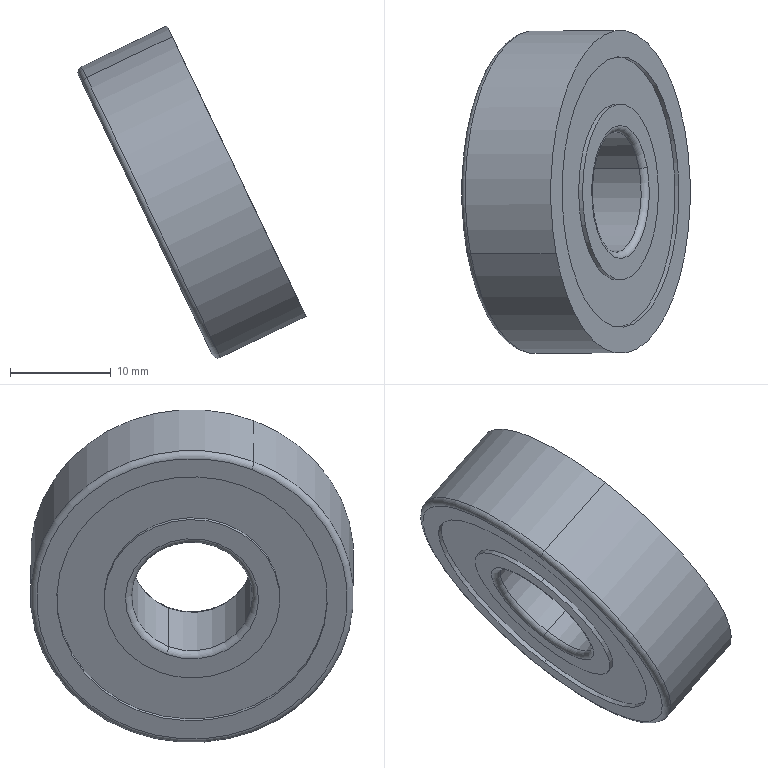Component | SolidWorks | AHTF30S5M100-1_bearingB6201ZZ-1 | 1 solid | 24 faces | volume 6615 mm3 | cylinder 12 | torus 6 | plane 6 | commonest cylinder face diameters 26.8 x4 17.4 x4 12 x2 32 x2
build123d program:
from build123d import *


with BuildPart() as part:
    # Sketch1 → Revolve1 (revolve)
    with BuildSketch(Plane.XY, mode=Mode.PRIVATE) as revolve1_sk:
        with BuildLine():
            Line((0, 16), (0, 13.4))
            Line((0, 13.4), (0.433, 13.4))
            Line((0.433, 13.4), (0.433, 8.7))
            Line((0.433, 8.7), (0, 8.7))
            Line((0, 8.7), (0, 6.6))
            ThreePointArc((0, 6.6), (0.1757, 6.176), (0.6, 6))
            Line((0.6, 6), (9.4, 6))
            ThreePointArc((9.4, 6), (9.824, 6.176), (10, 6.6))
            Line((10, 6.6), (10, 8.7))
            Line((10, 8.7), (9.567, 8.7))
            Line((9.567, 8.7), (9.567, 13.4))
            Line((9.567, 13.4), (10, 13.4))
            Line((10, 13.4), (10, 15.4))
            ThreePointArc((10, 15.4), (9.824, 15.824), (9.4, 16))
            Line((9.4, 16), (0, 16))
        make_face()
    revolve(revolve1_sk.sketch.rotate(Axis((10, 0, 0), (-1, 0, 0)), 270), axis=Axis((10, 0, 0), (-1, 0, 0)))


solid = part.part

# Placed as in the assembly
solid = solid.moved(Location((4.018, 250, 460.302), (47.482, -17.927, -161.443)))
STEP:
#1=COLOUR_RGB('',0.7922,0.8196,0.9333);
#2=FILL_AREA_STYLE_COLOUR('',#1);
#3=FILL_AREA_STYLE('',(#2));
#4=SURFACE_STYLE_FILL_AREA(#3);
#5=SURFACE_SIDE_STYLE('',(#4));
#6=SURFACE_STYLE_USAGE(.BOTH.,#5);
#7=PRESENTATION_STYLE_ASSIGNMENT((#6));
#8=CARTESIAN_POINT('',(0.04487,10.075,17.447));
#9=VERTEX_POINT('',#8);
#10=CARTESIAN_POINT('',(-0.4387,9.61,18.457));
#11=VERTEX_POINT('',#10);
#12=CARTESIAN_POINT('',(-0.1969,9.843,17.952));
#13=DIRECTION('',(0.902,-0.,0.4318));
#14=DIRECTION('',(0.3988,0.3832,-0.8331));
#15=AXIS2_PLACEMENT_3D('',#12,#13,#14);
#16=CIRCLE('',#15,0.6063);
#17=EDGE_CURVE('',#9,#11,#16,.T.);
#18=ORIENTED_EDGE('',*,*,#17,.T.);
#19=CARTESIAN_POINT('',(-0.4269,9.601,18.487));
#20=VERTEX_POINT('',#19);
#21=CARTESIAN_POINT('',(-0.4174,9.61,18.467));
#22=DIRECTION('',(-0.1654,0.9237,0.3456));
#23=DIRECTION('',(0.,-0.3504,0.9366));
#24=AXIS2_PLACEMENT_3D('',#21,#22,#23);
#25=CIRCLE('',#24,0.02362);
#26=EDGE_CURVE('',#11,#20,#25,.T.);
#27=ORIENTED_EDGE('',*,*,#26,.T.);
#28=CARTESIAN_POINT('',(0.0756,10.084,17.438));
#29=VERTEX_POINT('',#28);
#30=CARTESIAN_POINT('',(-0.1756,9.843,17.962));
#31=DIRECTION('',(0.902,-0.,0.4318));
#32=DIRECTION('',(0.3988,0.3832,-0.8331));
#33=AXIS2_PLACEMENT_3D('',#30,#31,#32);
#34=CIRCLE('',#33,0.6299);
#35=EDGE_CURVE('',#29,#20,#34,.T.);
#36=ORIENTED_EDGE('',*,*,#35,.F.);
#37=CARTESIAN_POINT('',(0.06618,10.075,17.457));
#38=DIRECTION('',(0.1654,-0.9237,-0.3456));
#39=DIRECTION('',(0.,0.3504,-0.9366));
#40=AXIS2_PLACEMENT_3D('',#37,#38,#39);
#41=CIRCLE('',#40,0.02362);
#42=EDGE_CURVE('',#9,#29,#41,.T.);
#43=ORIENTED_EDGE('',*,*,#42,.F.);
#44=EDGE_LOOP('',(#18,#27,#36,#43));
#45=FACE_OUTER_BOUND('',#44,.T.);
#46=CARTESIAN_POINT('',(-0.1756,9.843,17.962));
#47=DIRECTION('',(0.902,-0.,0.4318));
#48=DIRECTION('',(0.3988,0.3832,-0.8331));
#49=AXIS2_PLACEMENT_3D('',#46,#47,#48);
#50=TOROIDAL_SURFACE('',#49,0.6063,0.02362);
#51=ADVANCED_FACE('',(#45),#50,.T.);
#52=CARTESIAN_POINT('',(-0.4073,9.64,18.392));
#53=VERTEX_POINT('',#52);
#54=CARTESIAN_POINT('',(0.01347,10.045,17.513));
#55=VERTEX_POINT('',#54);
#56=CARTESIAN_POINT('',(-0.1969,9.843,17.952));
#57=DIRECTION('',(0.902,-0.,0.4318));
#58=DIRECTION('',(0.3988,0.3832,-0.8331));
#59=AXIS2_PLACEMENT_3D('',#56,#57,#58);
#60=CIRCLE('',#59,0.5276);
#61=EDGE_CURVE('',#53,#55,#60,.T.);
#62=ORIENTED_EDGE('',*,*,#61,.F.);
#63=CARTESIAN_POINT('',(-0.392,9.64,18.399));
#64=VERTEX_POINT('',#63);
#65=CARTESIAN_POINT('',(-0.4073,9.64,18.392));
#66=DIRECTION('',(0.902,-0.,0.4318));
#67=VECTOR('',#66,39.37);
#68=LINE('',#65,#67);
#69=EDGE_CURVE('',#53,#64,#68,.T.);
#70=ORIENTED_EDGE('',*,*,#69,.T.);
#71=CARTESIAN_POINT('',(0.02884,10.045,17.52));
#72=VERTEX_POINT('',#71);
#73=CARTESIAN_POINT('',(-0.1816,9.843,17.959));
#74=DIRECTION('',(0.902,-0.,0.4318));
#75=DIRECTION('',(0.3988,0.3832,-0.8331));
#76=AXIS2_PLACEMENT_3D('',#73,#74,#75);
#77=CIRCLE('',#76,0.5276);
#78=EDGE_CURVE('',#64,#72,#77,.T.);
#79=ORIENTED_EDGE('',*,*,#78,.T.);
#80=CARTESIAN_POINT('',(0.01347,10.045,17.513));
#81=DIRECTION('',(0.902,-0.,0.4318));
#82=VECTOR('',#81,39.37);
#83=LINE('',#80,#82);
#84=EDGE_CURVE('',#55,#72,#83,.T.);
#85=ORIENTED_EDGE('',*,*,#84,.F.);
#86=EDGE_LOOP('',(#62,#70,#79,#85));
#87=FACE_OUTER_BOUND('',#86,.T.);
#88=CARTESIAN_POINT('',(-0.1969,9.843,17.952));
#89=DIRECTION('',(0.902,-0.,0.4318));
#90=DIRECTION('',(0.3988,0.3832,-0.8331));
#91=AXIS2_PLACEMENT_3D('',#88,#89,#90);
#92=CYLINDRICAL_SURFACE('',#91,0.5276);
#93=ADVANCED_FACE('',(#87),#92,.F.);
#94=CARTESIAN_POINT('',(-0.06033,9.974,17.667));
#95=VERTEX_POINT('',#94);
#96=CARTESIAN_POINT('',(-0.3335,9.711,18.237));
#97=VERTEX_POINT('',#96);
#98=CARTESIAN_POINT('',(-0.1969,9.843,17.952));
#99=DIRECTION('',(0.902,-0.,0.4318));
#100=DIRECTION('',(0.3988,0.3832,-0.8331));
#101=AXIS2_PLACEMENT_3D('',#98,#99,#100);
#102=CIRCLE('',#101,0.3425);
#103=EDGE_CURVE('',#95,#97,#102,.T.);
#104=ORIENTED_EDGE('',*,*,#103,.T.);
#105=CARTESIAN_POINT('',(-0.3182,9.711,18.245));
#106=VERTEX_POINT('',#105);
#107=CARTESIAN_POINT('',(-0.3335,9.711,18.237));
#108=DIRECTION('',(0.902,-0.,0.4318));
#109=VECTOR('',#108,39.37);
#110=LINE('',#107,#109);
#111=EDGE_CURVE('',#97,#106,#110,.T.);
#112=ORIENTED_EDGE('',*,*,#111,.T.);
#113=CARTESIAN_POINT('',(-0.04496,9.974,17.674));
#114=VERTEX_POINT('',#113);
#115=CARTESIAN_POINT('',(-0.1816,9.843,17.959));
#116=DIRECTION('',(0.902,-0.,0.4318));
#117=DIRECTION('',(0.3988,0.3832,-0.8331));
#118=AXIS2_PLACEMENT_3D('',#115,#116,#117);
#119=CIRCLE('',#118,0.3425);
#120=EDGE_CURVE('',#114,#106,#119,.T.);
#121=ORIENTED_EDGE('',*,*,#120,.F.);
#122=CARTESIAN_POINT('',(-0.06033,9.974,17.667));
#123=DIRECTION('',(0.902,-0.,0.4318));
#124=VECTOR('',#123,39.37);
#125=LINE('',#122,#124);
#126=EDGE_CURVE('',#95,#114,#125,.T.);
#127=ORIENTED_EDGE('',*,*,#126,.F.);
#128=EDGE_LOOP('',(#104,#112,#121,#127));
#129=FACE_OUTER_BOUND('',#128,.T.);
#130=CARTESIAN_POINT('',(-0.1969,9.843,17.952));
#131=DIRECTION('',(0.902,-0.,0.4318));
#132=DIRECTION('',(0.3988,0.3832,-0.8331));
#133=AXIS2_PLACEMENT_3D('',#130,#131,#132);
#134=CYLINDRICAL_SURFACE('',#133,0.3425);
#135=ADVANCED_FACE('',(#129),#134,.T.);
#136=CARTESIAN_POINT('',(-0.08142,9.933,17.766));
#137=VERTEX_POINT('',#136);
#138=CARTESIAN_POINT('',(-0.2698,9.752,18.159));
#139=VERTEX_POINT('',#138);
#140=CARTESIAN_POINT('',(-0.1756,9.843,17.962));
#141=DIRECTION('',(0.902,-0.,0.4318));
#142=DIRECTION('',(0.3988,0.3832,-0.8331));
#143=AXIS2_PLACEMENT_3D('',#140,#141,#142);
#144=CIRCLE('',#143,0.2362);
#145=EDGE_CURVE('',#137,#139,#144,.T.);
#146=ORIENTED_EDGE('',*,*,#145,.T.);
#147=CARTESIAN_POINT('',(-0.3006,9.743,18.169));
#148=VERTEX_POINT('',#147);
#149=CARTESIAN_POINT('',(-0.2793,9.743,18.179));
#150=DIRECTION('',(-0.1654,0.9237,0.3456));
#151=DIRECTION('',(0.,-0.3504,0.9366));
#152=AXIS2_PLACEMENT_3D('',#149,#150,#151);
#153=CIRCLE('',#152,0.02362);
#154=EDGE_CURVE('',#139,#148,#153,.T.);
#155=ORIENTED_EDGE('',*,*,#154,.T.);
#156=CARTESIAN_POINT('',(-0.09331,9.942,17.736));
#157=VERTEX_POINT('',#156);
#158=CARTESIAN_POINT('',(-0.1969,9.843,17.952));
#159=DIRECTION('',(0.902,-0.,0.4318));
#160=DIRECTION('',(0.3988,0.3832,-0.8331));
#161=AXIS2_PLACEMENT_3D('',#158,#159,#160);
#162=CIRCLE('',#161,0.2598);
#163=EDGE_CURVE('',#157,#148,#162,.T.);
#164=ORIENTED_EDGE('',*,*,#163,.F.);
#165=CARTESIAN_POINT('',(-0.072,9.942,17.746));
#166=DIRECTION('',(0.1654,-0.9237,-0.3456));
#167=DIRECTION('',(0.,0.3504,-0.9366));
#168=AXIS2_PLACEMENT_3D('',#165,#166,#167);
#169=CIRCLE('',#168,0.02362);
#170=EDGE_CURVE('',#137,#157,#169,.T.);
#171=ORIENTED_EDGE('',*,*,#170,.F.);
#172=EDGE_LOOP('',(#146,#155,#164,#171));
#173=FACE_OUTER_BOUND('',#172,.T.);
#174=CARTESIAN_POINT('',(-0.1756,9.843,17.962));
#175=DIRECTION('',(0.902,-0.,0.4318));
#176=DIRECTION('',(0.3988,0.3832,-0.8331));
#177=AXIS2_PLACEMENT_3D('',#174,#175,#176);
#178=TOROIDAL_SURFACE('',#177,0.2598,0.02362);
#179=ADVANCED_FACE('',(#173),#178,.T.);
#180=CARTESIAN_POINT('',(-0.1756,9.843,17.962));
#181=DIRECTION('',(0.902,-0.,0.4318));
#182=DIRECTION('',(0.3988,0.3832,-0.8331));
#183=AXIS2_PLACEMENT_3D('',#180,#181,#182);
#184=CIRCLE('',#183,0.2362);
#185=EDGE_CURVE('',#139,#137,#184,.T.);
#186=ORIENTED_EDGE('',*,*,#185,.F.);
#187=CARTESIAN_POINT('',(0.04265,9.752,18.309));
#188=VERTEX_POINT('',#187);
#189=CARTESIAN_POINT('',(-0.2912,9.752,18.149));
#190=DIRECTION('',(0.902,-0.,0.4318));
#191=VECTOR('',#190,39.37);
#192=LINE('',#189,#191);
#193=EDGE_CURVE('',#139,#188,#192,.T.);
#194=ORIENTED_EDGE('',*,*,#193,.T.);
#195=CARTESIAN_POINT('',(0.2311,9.933,17.915));
#196=VERTEX_POINT('',#195);
#197=CARTESIAN_POINT('',(0.1369,9.843,18.112));
#198=DIRECTION('',(0.902,-0.,0.4318));
#199=DIRECTION('',(0.3988,0.3832,-0.8331));
#200=AXIS2_PLACEMENT_3D('',#197,#198,#199);
#201=CIRCLE('',#200,0.2362);
#202=EDGE_CURVE('',#188,#196,#201,.T.);
#203=ORIENTED_EDGE('',*,*,#202,.T.);
#204=CARTESIAN_POINT('',(-0.1027,9.933,17.755));
#205=DIRECTION('',(0.902,-0.,0.4318));
#206=VECTOR('',#205,39.37);
#207=LINE('',#204,#206);
#208=EDGE_CURVE('',#137,#196,#207,.T.);
#209=ORIENTED_EDGE('',*,*,#208,.F.);
#210=EDGE_LOOP('',(#186,#194,#203,#209));
#211=FACE_OUTER_BOUND('',#210,.T.);
#212=CARTESIAN_POINT('',(-0.1969,9.843,17.952));
#213=DIRECTION('',(0.902,-0.,0.4318));
#214=DIRECTION('',(0.3988,0.3832,-0.8331));
#215=AXIS2_PLACEMENT_3D('',#212,#213,#214);
#216=CYLINDRICAL_SURFACE('',#215,0.2362);
#217=ADVANCED_FACE('',(#211),#216,.F.);
#218=CARTESIAN_POINT('',(0.2618,9.942,17.906));
#219=VERTEX_POINT('',#218);
#220=CARTESIAN_POINT('',(0.05454,9.743,18.339));
#221=VERTEX_POINT('',#220);
#222=CARTESIAN_POINT('',(0.1582,9.843,18.122));
#223=DIRECTION('',(0.902,-0.,0.4318));
#224=DIRECTION('',(0.3988,0.3832,-0.8331));
#225=AXIS2_PLACEMENT_3D('',#222,#223,#224);
#226=CIRCLE('',#225,0.2598);
#227=EDGE_CURVE('',#219,#221,#226,.T.);
#228=ORIENTED_EDGE('',*,*,#227,.T.);
#229=CARTESIAN_POINT('',(0.03323,9.743,18.328));
#230=DIRECTION('',(-0.1654,0.9237,0.3456));
#231=DIRECTION('',(0.,-0.3504,0.9366));
#232=AXIS2_PLACEMENT_3D('',#229,#230,#231);
#233=CIRCLE('',#232,0.02362);
#234=EDGE_CURVE('',#221,#188,#233,.T.);
#235=ORIENTED_EDGE('',*,*,#234,.T.);
#236=CARTESIAN_POINT('',(0.1369,9.843,18.112));
#237=DIRECTION('',(0.902,-0.,0.4318));
#238=DIRECTION('',(0.3988,0.3832,-0.8331));
#239=AXIS2_PLACEMENT_3D('',#236,#237,#238);
#240=CIRCLE('',#239,0.2362);
#241=EDGE_CURVE('',#196,#188,#240,.T.);
#242=ORIENTED_EDGE('',*,*,#241,.F.);
#243=CARTESIAN_POINT('',(0.2405,9.942,17.895));
#244=DIRECTION('',(0.1654,-0.9237,-0.3456));
#245=DIRECTION('',(0.,0.3504,-0.9366));
#246=AXIS2_PLACEMENT_3D('',#243,#244,#245);
#247=CIRCLE('',#246,0.02362);
#248=EDGE_CURVE('',#219,#196,#247,.T.);
#249=ORIENTED_EDGE('',*,*,#248,.F.);
#250=EDGE_LOOP('',(#228,#235,#242,#249));
#251=FACE_OUTER_BOUND('',#250,.T.);
#252=CARTESIAN_POINT('',(0.1369,9.843,18.112));
#253=DIRECTION('',(0.902,-0.,0.4318));
#254=DIRECTION('',(0.3988,0.3832,-0.8331));
#255=AXIS2_PLACEMENT_3D('',#252,#253,#254);
#256=TOROIDAL_SURFACE('',#255,0.2598,0.02362);
#257=ADVANCED_FACE('',(#251),#256,.T.);
#258=CARTESIAN_POINT('',(0.2794,9.974,17.829));
#259=VERTEX_POINT('',#258);
#260=CARTESIAN_POINT('',(0.006187,9.711,18.4));
#261=VERTEX_POINT('',#260);
#262=CARTESIAN_POINT('',(0.1428,9.843,18.115));
#263=DIRECTION('',(0.902,-0.,0.4318));
#264=DIRECTION('',(0.3988,0.3832,-0.8331));
#265=AXIS2_PLACEMENT_3D('',#262,#263,#264);
#266=CIRCLE('',#265,0.3425);
#267=EDGE_CURVE('',#259,#261,#266,.T.);
#268=ORIENTED_EDGE('',*,*,#267,.T.);
#269=CARTESIAN_POINT('',(0.02156,9.711,18.407));
#270=VERTEX_POINT('',#269);
#271=CARTESIAN_POINT('',(-0.3335,9.711,18.237));
#272=DIRECTION('',(0.902,-0.,0.4318));
#273=VECTOR('',#272,39.37);
#274=LINE('',#271,#273);
#275=EDGE_CURVE('',#261,#270,#274,.T.);
#276=ORIENTED_EDGE('',*,*,#275,.T.);
#277=CARTESIAN_POINT('',(0.2948,9.974,17.837));
#278=VERTEX_POINT('',#277);
#279=CARTESIAN_POINT('',(0.1582,9.843,18.122));
#280=DIRECTION('',(0.902,-0.,0.4318));
#281=DIRECTION('',(0.3988,0.3832,-0.8331));
#282=AXIS2_PLACEMENT_3D('',#279,#280,#281);
#283=CIRCLE('',#282,0.3425);
#284=EDGE_CURVE('',#278,#270,#283,.T.);
#285=ORIENTED_EDGE('',*,*,#284,.F.);
#286=CARTESIAN_POINT('',(-0.06033,9.974,17.667));
#287=DIRECTION('',(0.902,-0.,0.4318));
#288=VECTOR('',#287,39.37);
#289=LINE('',#286,#288);
#290=EDGE_CURVE('',#259,#278,#289,.T.);
#291=ORIENTED_EDGE('',*,*,#290,.F.);
#292=EDGE_LOOP('',(#268,#276,#285,#291));
#293=FACE_OUTER_BOUND('',#292,.T.);
#294=CARTESIAN_POINT('',(-0.1969,9.843,17.952));
#295=DIRECTION('',(0.902,-0.,0.4318));
#296=DIRECTION('',(0.3988,0.3832,-0.8331));
#297=AXIS2_PLACEMENT_3D('',#294,#295,#296);
#298=CYLINDRICAL_SURFACE('',#297,0.3425);
#299=ADVANCED_FACE('',(#293),#298,.T.);
#300=CARTESIAN_POINT('',(-0.06761,9.64,18.554));
#301=VERTEX_POINT('',#300);
#302=CARTESIAN_POINT('',(0.3532,10.045,17.675));
#303=VERTEX_POINT('',#302);
#304=CARTESIAN_POINT('',(0.1428,9.843,18.115));
#305=DIRECTION('',(0.902,-0.,0.4318));
#306=DIRECTION('',(0.3988,0.3832,-0.8331));
#307=AXIS2_PLACEMENT_3D('',#304,#305,#306);
#308=CIRCLE('',#307,0.5276);
#309=EDGE_CURVE('',#301,#303,#308,.T.);
#310=ORIENTED_EDGE('',*,*,#309,.F.);
#311=CARTESIAN_POINT('',(-0.05224,9.64,18.562));
#312=VERTEX_POINT('',#311);
#313=CARTESIAN_POINT('',(-0.4073,9.64,18.392));
#314=DIRECTION('',(0.902,-0.,0.4318));
#315=VECTOR('',#314,39.37);
#316=LINE('',#313,#315);
#317=EDGE_CURVE('',#301,#312,#316,.T.);
#318=ORIENTED_EDGE('',*,*,#317,.T.);
#319=CARTESIAN_POINT('',(0.3686,10.045,17.683));
#320=VERTEX_POINT('',#319);
#321=CARTESIAN_POINT('',(0.1582,9.843,18.122));
#322=DIRECTION('',(0.902,-0.,0.4318));
#323=DIRECTION('',(0.3988,0.3832,-0.8331));
#324=AXIS2_PLACEMENT_3D('',#321,#322,#323);
#325=CIRCLE('',#324,0.5276);
#326=EDGE_CURVE('',#312,#320,#325,.T.);
#327=ORIENTED_EDGE('',*,*,#326,.T.);
#328=CARTESIAN_POINT('',(0.01347,10.045,17.513));
#329=DIRECTION('',(0.902,-0.,0.4318));
#330=VECTOR('',#329,39.37);
#331=LINE('',#328,#330);
#332=EDGE_CURVE('',#303,#320,#331,.T.);
#333=ORIENTED_EDGE('',*,*,#332,.F.);
#334=EDGE_LOOP('',(#310,#318,#327,#333));
#335=FACE_OUTER_BOUND('',#334,.T.);
#336=CARTESIAN_POINT('',(-0.1969,9.843,17.952));
#337=DIRECTION('',(0.902,-0.,0.4318));
#338=DIRECTION('',(0.3988,0.3832,-0.8331));
#339=AXIS2_PLACEMENT_3D('',#336,#337,#338);
#340=CYLINDRICAL_SURFACE('',#339,0.5276);
#341=ADVANCED_FACE('',(#335),#340,.F.);
#342=ORIENTED_EDGE('',*,*,#35,.T.);
#343=CARTESIAN_POINT('',(-0.09306,9.601,18.647));
#344=VERTEX_POINT('',#343);
#345=CARTESIAN_POINT('',(-0.4482,9.601,18.477));
#346=DIRECTION('',(0.902,-0.,0.4318));
#347=VECTOR('',#346,39.37);
#348=LINE('',#345,#347);
#349=EDGE_CURVE('',#20,#344,#348,.T.);
#350=ORIENTED_EDGE('',*,*,#349,.T.);
#351=CARTESIAN_POINT('',(0.4094,10.084,17.597));
#352=VERTEX_POINT('',#351);
#353=CARTESIAN_POINT('',(0.1582,9.843,18.122));
#354=DIRECTION('',(0.902,-0.,0.4318));
#355=DIRECTION('',(0.3988,0.3832,-0.8331));
#356=AXIS2_PLACEMENT_3D('',#353,#354,#355);
#357=CIRCLE('',#356,0.6299);
#358=EDGE_CURVE('',#352,#344,#357,.T.);
#359=ORIENTED_EDGE('',*,*,#358,.F.);
#360=CARTESIAN_POINT('',(0.05429,10.084,17.427));
#361=DIRECTION('',(0.902,-0.,0.4318));
#362=VECTOR('',#361,39.37);
#363=LINE('',#360,#362);
#364=EDGE_CURVE('',#29,#352,#363,.T.);
#365=ORIENTED_EDGE('',*,*,#364,.F.);
#366=EDGE_LOOP('',(#342,#350,#359,#365));
#367=FACE_OUTER_BOUND('',#366,.T.);
#368=CARTESIAN_POINT('',(-0.1969,9.843,17.952));
#369=DIRECTION('',(0.902,-0.,0.4318));
#370=DIRECTION('',(0.3988,0.3832,-0.8331));
#371=AXIS2_PLACEMENT_3D('',#368,#369,#370);
#372=CYLINDRICAL_SURFACE('',#371,0.6299);
#373=ADVANCED_FACE('',(#367),#372,.T.);
#374=ORIENTED_EDGE('',*,*,#349,.F.);
#375=CARTESIAN_POINT('',(-0.1756,9.843,17.962));
#376=DIRECTION('',(0.902,-0.,0.4318));
#377=DIRECTION('',(0.3988,0.3832,-0.8331));
#378=AXIS2_PLACEMENT_3D('',#375,#376,#377);
#379=CIRCLE('',#378,0.6299);
#380=EDGE_CURVE('',#20,#29,#379,.T.);
#381=ORIENTED_EDGE('',*,*,#380,.T.);
#382=ORIENTED_EDGE('',*,*,#364,.T.);
#383=CARTESIAN_POINT('',(0.1582,9.843,18.122));
#384=DIRECTION('',(0.902,-0.,0.4318));
#385=DIRECTION('',(0.3988,0.3832,-0.8331));
#386=AXIS2_PLACEMENT_3D('',#383,#384,#385);
#387=CIRCLE('',#386,0.6299);
#388=EDGE_CURVE('',#344,#352,#387,.T.);
#389=ORIENTED_EDGE('',*,*,#388,.F.);
#390=EDGE_LOOP('',(#374,#381,#382,#389));
#391=FACE_OUTER_BOUND('',#390,.T.);
#392=CARTESIAN_POINT('',(-0.1969,9.843,17.952));
#393=DIRECTION('',(0.902,-0.,0.4318));
#394=DIRECTION('',(0.3988,0.3832,-0.8331));
#395=AXIS2_PLACEMENT_3D('',#392,#393,#394);
#396=CYLINDRICAL_SURFACE('',#395,0.6299);
#397=ADVANCED_FACE('',(#391),#396,.T.);
#398=CARTESIAN_POINT('',(0.1582,9.843,18.122));
#399=DIRECTION('',(0.902,-0.,0.4318));
#400=DIRECTION('',(0.3988,0.3832,-0.8331));
#401=AXIS2_PLACEMENT_3D('',#398,#399,#400);
#402=CIRCLE('',#401,0.5276);
#403=EDGE_CURVE('',#320,#312,#402,.T.);
#404=ORIENTED_EDGE('',*,*,#403,.F.);
#405=ORIENTED_EDGE('',*,*,#326,.F.);
#406=EDGE_LOOP('',(#404,#405));
#407=FACE_BOUND('',#406,.T.);
#408=ORIENTED_EDGE('',*,*,#358,.T.);
#409=ORIENTED_EDGE('',*,*,#388,.T.);
#410=EDGE_LOOP('',(#408,#409));
#411=FACE_OUTER_BOUND('',#410,.T.);
#412=CARTESIAN_POINT('',(0.05395,10.424,18.34));
#413=DIRECTION('',(-0.902,0.,-0.4318));
#414=DIRECTION('',(-0.3988,-0.3832,0.8331));
#415=AXIS2_PLACEMENT_3D('',#412,#413,#414);
#416=PLANE('',#415);
#417=ADVANCED_FACE('',(#407,#411),#416,.F.);
#418=ORIENTED_EDGE('',*,*,#317,.F.);
#419=CARTESIAN_POINT('',(0.1428,9.843,18.115));
#420=DIRECTION('',(0.902,-0.,0.4318));
#421=DIRECTION('',(0.3988,0.3832,-0.8331));
#422=AXIS2_PLACEMENT_3D('',#419,#420,#421);
#423=CIRCLE('',#422,0.5276);
#424=EDGE_CURVE('',#303,#301,#423,.T.);
#425=ORIENTED_EDGE('',*,*,#424,.F.);
#426=ORIENTED_EDGE('',*,*,#332,.T.);
#427=ORIENTED_EDGE('',*,*,#403,.T.);
#428=EDGE_LOOP('',(#418,#425,#426,#427));
#429=FACE_OUTER_BOUND('',#428,.T.);
#430=CARTESIAN_POINT('',(-0.1969,9.843,17.952));
#431=DIRECTION('',(0.902,-0.,0.4318));
#432=DIRECTION('',(0.3988,0.3832,-0.8331));
#433=AXIS2_PLACEMENT_3D('',#430,#431,#432);
#434=CYLINDRICAL_SURFACE('',#433,0.5276);
#435=ADVANCED_FACE('',(#429),#434,.F.);
#436=ORIENTED_EDGE('',*,*,#267,.F.);
#437=CARTESIAN_POINT('',(0.1428,9.843,18.115));
#438=DIRECTION('',(0.902,-0.,0.4318));
#439=DIRECTION('',(0.3988,0.3832,-0.8331));
#440=AXIS2_PLACEMENT_3D('',#437,#438,#439);
#441=CIRCLE('',#440,0.3425);
#442=EDGE_CURVE('',#261,#259,#441,.T.);
#443=ORIENTED_EDGE('',*,*,#442,.F.);
#444=EDGE_LOOP('',(#436,#443));
#445=FACE_BOUND('',#444,.T.);
#446=ORIENTED_EDGE('',*,*,#424,.T.);
#447=ORIENTED_EDGE('',*,*,#309,.T.);
#448=EDGE_LOOP('',(#446,#447));
#449=FACE_OUTER_BOUND('',#448,.T.);
#450=CARTESIAN_POINT('',(0.05551,10.33,18.297));
#451=DIRECTION('',(-0.902,0.,-0.4318));
#452=DIRECTION('',(-0.3988,-0.3832,0.8331));
#453=AXIS2_PLACEMENT_3D('',#450,#451,#452);
#454=PLANE('',#453);
#455=ADVANCED_FACE('',(#445,#449),#454,.F.);
#456=ORIENTED_EDGE('',*,*,#275,.F.);
#457=ORIENTED_EDGE('',*,*,#442,.T.);
#458=ORIENTED_EDGE('',*,*,#290,.T.);
#459=CARTESIAN_POINT('',(0.1582,9.843,18.122));
#460=DIRECTION('',(0.902,-0.,0.4318));
#461=DIRECTION('',(0.3988,0.3832,-0.8331));
#462=AXIS2_PLACEMENT_3D('',#459,#460,#461);
#463=CIRCLE('',#462,0.3425);
#464=EDGE_CURVE('',#270,#278,#463,.T.);
#465=ORIENTED_EDGE('',*,*,#464,.F.);
#466=EDGE_LOOP('',(#456,#457,#458,#465));
#467=FACE_OUTER_BOUND('',#466,.T.);
#468=CARTESIAN_POINT('',(-0.1969,9.843,17.952));
#469=DIRECTION('',(0.902,-0.,0.4318));
#470=DIRECTION('',(0.3988,0.3832,-0.8331));
#471=AXIS2_PLACEMENT_3D('',#468,#469,#470);
#472=CYLINDRICAL_SURFACE('',#471,0.3425);
#473=ADVANCED_FACE('',(#467),#472,.T.);
#474=ORIENTED_EDGE('',*,*,#227,.F.);
#475=CARTESIAN_POINT('',(0.1582,9.843,18.122));
#476=DIRECTION('',(0.902,-0.,0.4318));
#477=DIRECTION('',(0.3988,0.3832,-0.8331));
#478=AXIS2_PLACEMENT_3D('',#475,#476,#477);
#479=CIRCLE('',#478,0.2598);
#480=EDGE_CURVE('',#221,#219,#479,.T.);
#481=ORIENTED_EDGE('',*,*,#480,.F.);
#482=EDGE_LOOP('',(#474,#481));
#483=FACE_BOUND('',#482,.T.);
#484=ORIENTED_EDGE('',*,*,#284,.T.);
#485=ORIENTED_EDGE('',*,*,#464,.T.);
#486=EDGE_LOOP('',(#484,#485));
#487=FACE_OUTER_BOUND('',#486,.T.);
#488=CARTESIAN_POINT('',(0.1015,10.159,18.24));
#489=DIRECTION('',(-0.902,0.,-0.4318));
#490=DIRECTION('',(-0.3988,-0.3832,0.8331));
#491=AXIS2_PLACEMENT_3D('',#488,#489,#490);
#492=PLANE('',#491);
#493=ADVANCED_FACE('',(#483,#487),#492,.F.);
#494=ORIENTED_EDGE('',*,*,#234,.F.);
#495=ORIENTED_EDGE('',*,*,#480,.T.);
#496=ORIENTED_EDGE('',*,*,#248,.T.);
#497=ORIENTED_EDGE('',*,*,#202,.F.);
#498=EDGE_LOOP('',(#494,#495,#496,#497));
#499=FACE_OUTER_BOUND('',#498,.T.);
#500=CARTESIAN_POINT('',(0.1369,9.843,18.112));
#501=DIRECTION('',(0.902,-0.,0.4318));
#502=DIRECTION('',(0.3988,0.3832,-0.8331));
#503=AXIS2_PLACEMENT_3D('',#500,#501,#502);
#504=TOROIDAL_SURFACE('',#503,0.2598,0.02362);
#505=ADVANCED_FACE('',(#499),#504,.T.);
#506=ORIENTED_EDGE('',*,*,#193,.F.);
#507=ORIENTED_EDGE('',*,*,#145,.F.);
#508=ORIENTED_EDGE('',*,*,#208,.T.);
#509=ORIENTED_EDGE('',*,*,#241,.T.);
#510=EDGE_LOOP('',(#506,#507,#508,#509));
#511=FACE_OUTER_BOUND('',#510,.T.);
#512=CARTESIAN_POINT('',(-0.1969,9.843,17.952));
#513=DIRECTION('',(0.902,-0.,0.4318));
#514=DIRECTION('',(0.3988,0.3832,-0.8331));
#515=AXIS2_PLACEMENT_3D('',#512,#513,#514);
#516=CYLINDRICAL_SURFACE('',#515,0.2362);
#517=ADVANCED_FACE('',(#511),#516,.F.);
#518=ORIENTED_EDGE('',*,*,#154,.F.);
#519=ORIENTED_EDGE('',*,*,#185,.T.);
#520=ORIENTED_EDGE('',*,*,#170,.T.);
#521=CARTESIAN_POINT('',(-0.1969,9.843,17.952));
#522=DIRECTION('',(0.902,-0.,0.4318));
#523=DIRECTION('',(0.3988,0.3832,-0.8331));
#524=AXIS2_PLACEMENT_3D('',#521,#522,#523);
#525=CIRCLE('',#524,0.2598);
#526=EDGE_CURVE('',#148,#157,#525,.T.);
#527=ORIENTED_EDGE('',*,*,#526,.F.);
#528=EDGE_LOOP('',(#518,#519,#520,#527));
#529=FACE_OUTER_BOUND('',#528,.T.);
#530=CARTESIAN_POINT('',(-0.1756,9.843,17.962));
#531=DIRECTION('',(0.902,-0.,0.4318));
#532=DIRECTION('',(0.3988,0.3832,-0.8331));
#533=AXIS2_PLACEMENT_3D('',#530,#531,#532);
#534=TOROIDAL_SURFACE('',#533,0.2598,0.02362);
#535=ADVANCED_FACE('',(#529),#534,.T.);
#536=ORIENTED_EDGE('',*,*,#103,.F.);
#537=CARTESIAN_POINT('',(-0.1969,9.843,17.952));
#538=DIRECTION('',(0.902,-0.,0.4318));
#539=DIRECTION('',(0.3988,0.3832,-0.8331));
#540=AXIS2_PLACEMENT_3D('',#537,#538,#539);
#541=CIRCLE('',#540,0.3425);
#542=EDGE_CURVE('',#97,#95,#541,.T.);
#543=ORIENTED_EDGE('',*,*,#542,.F.);
#544=EDGE_LOOP('',(#536,#543));
#545=FACE_OUTER_BOUND('',#544,.T.);
#546=ORIENTED_EDGE('',*,*,#163,.T.);
#547=ORIENTED_EDGE('',*,*,#526,.T.);
#548=EDGE_LOOP('',(#546,#547));
#549=FACE_BOUND('',#548,.T.);
#550=CARTESIAN_POINT('',(-0.2399,10.083,18.042));
#551=DIRECTION('',(0.902,-0.,0.4318));
#552=DIRECTION('',(0.3988,0.3832,-0.8331));
#553=AXIS2_PLACEMENT_3D('',#550,#551,#552);
#554=PLANE('',#553);
#555=ADVANCED_FACE('',(#545,#549),#554,.F.);
#556=ORIENTED_EDGE('',*,*,#111,.F.);
#557=ORIENTED_EDGE('',*,*,#542,.T.);
#558=ORIENTED_EDGE('',*,*,#126,.T.);
#559=CARTESIAN_POINT('',(-0.1816,9.843,17.959));
#560=DIRECTION('',(0.902,-0.,0.4318));
#561=DIRECTION('',(0.3988,0.3832,-0.8331));
#562=AXIS2_PLACEMENT_3D('',#559,#560,#561);
#563=CIRCLE('',#562,0.3425);
#564=EDGE_CURVE('',#106,#114,#563,.T.);
#565=ORIENTED_EDGE('',*,*,#564,.F.);
#566=EDGE_LOOP('',(#556,#557,#558,#565));
#567=FACE_OUTER_BOUND('',#566,.T.);
#568=CARTESIAN_POINT('',(-0.1969,9.843,17.952));
#569=DIRECTION('',(0.902,-0.,0.4318));
#570=DIRECTION('',(0.3988,0.3832,-0.8331));
#571=AXIS2_PLACEMENT_3D('',#568,#569,#570);
#572=CYLINDRICAL_SURFACE('',#571,0.3425);
#573=ADVANCED_FACE('',(#567),#572,.T.);
#574=CARTESIAN_POINT('',(-0.1816,9.843,17.959));
#575=DIRECTION('',(0.902,-0.,0.4318));
#576=DIRECTION('',(0.3988,0.3832,-0.8331));
#577=AXIS2_PLACEMENT_3D('',#574,#575,#576);
#578=CIRCLE('',#577,0.5276);
#579=EDGE_CURVE('',#72,#64,#578,.T.);
#580=ORIENTED_EDGE('',*,*,#579,.F.);
#581=ORIENTED_EDGE('',*,*,#78,.F.);
#582=EDGE_LOOP('',(#580,#581));
#583=FACE_OUTER_BOUND('',#582,.T.);
#584=ORIENTED_EDGE('',*,*,#120,.T.);
#585=ORIENTED_EDGE('',*,*,#564,.T.);
#586=EDGE_LOOP('',(#584,#585));
#587=FACE_BOUND('',#586,.T.);
#588=CARTESIAN_POINT('',(-0.2382,10.159,18.078));
#589=DIRECTION('',(0.902,-0.,0.4318));
#590=DIRECTION('',(0.3988,0.3832,-0.8331));
#591=AXIS2_PLACEMENT_3D('',#588,#589,#590);
#592=PLANE('',#591);
#593=ADVANCED_FACE('',(#583,#587),#592,.F.);
#594=ORIENTED_EDGE('',*,*,#69,.F.);
#595=CARTESIAN_POINT('',(-0.1969,9.843,17.952));
#596=DIRECTION('',(0.902,-0.,0.4318));
#597=DIRECTION('',(0.3988,0.3832,-0.8331));
#598=AXIS2_PLACEMENT_3D('',#595,#596,#597);
#599=CIRCLE('',#598,0.5276);
#600=EDGE_CURVE('',#55,#53,#599,.T.);
#601=ORIENTED_EDGE('',*,*,#600,.F.);
#602=ORIENTED_EDGE('',*,*,#84,.T.);
#603=ORIENTED_EDGE('',*,*,#579,.T.);
#604=EDGE_LOOP('',(#594,#601,#602,#603));
#605=FACE_OUTER_BOUND('',#604,.T.);
#606=CARTESIAN_POINT('',(-0.1969,9.843,17.952));
#607=DIRECTION('',(0.902,-0.,0.4318));
#608=DIRECTION('',(0.3988,0.3832,-0.8331));
#609=AXIS2_PLACEMENT_3D('',#606,#607,#608);
#610=CYLINDRICAL_SURFACE('',#609,0.5276);
#611=ADVANCED_FACE('',(#605),#610,.F.);
#612=ORIENTED_EDGE('',*,*,#17,.F.);
#613=CARTESIAN_POINT('',(-0.1969,9.843,17.952));
#614=DIRECTION('',(0.902,-0.,0.4318));
#615=DIRECTION('',(0.3988,0.3832,-0.8331));
#616=AXIS2_PLACEMENT_3D('',#613,#614,#615);
#617=CIRCLE('',#616,0.6063);
#618=EDGE_CURVE('',#11,#9,#617,.T.);
#619=ORIENTED_EDGE('',*,*,#618,.F.);
#620=EDGE_LOOP('',(#612,#619));
#621=FACE_OUTER_BOUND('',#620,.T.);
#622=ORIENTED_EDGE('',*,*,#600,.T.);
#623=ORIENTED_EDGE('',*,*,#61,.T.);
#624=EDGE_LOOP('',(#622,#623));
#625=FACE_BOUND('',#624,.T.);
#626=CARTESIAN_POINT('',(-0.2842,10.33,18.134));
#627=DIRECTION('',(0.902,-0.,0.4318));
#628=DIRECTION('',(0.3988,0.3832,-0.8331));
#629=AXIS2_PLACEMENT_3D('',#626,#627,#628);
#630=PLANE('',#629);
#631=ADVANCED_FACE('',(#621,#625),#630,.F.);
#632=ORIENTED_EDGE('',*,*,#26,.F.);
#633=ORIENTED_EDGE('',*,*,#618,.T.);
#634=ORIENTED_EDGE('',*,*,#42,.T.);
#635=ORIENTED_EDGE('',*,*,#380,.F.);
#636=EDGE_LOOP('',(#632,#633,#634,#635));
#637=FACE_OUTER_BOUND('',#636,.T.);
#638=CARTESIAN_POINT('',(-0.1756,9.843,17.962));
#639=DIRECTION('',(0.902,-0.,0.4318));
#640=DIRECTION('',(0.3988,0.3832,-0.8331));
#641=AXIS2_PLACEMENT_3D('',#638,#639,#640);
#642=TOROIDAL_SURFACE('',#641,0.6063,0.02362);
#643=ADVANCED_FACE('',(#637),#642,.T.);
#644=CLOSED_SHELL('',(#51,#93,#135,#179,#217,#257,#299,#341,#373,#397,#417,#435,#455,#473,#493,#505,#517,#535,#555,#573,#593,#611,#631,#643));
#645=MANIFOLD_SOLID_BREP('',#644);
#646=STYLED_ITEM('',(#7),#645);
#647=(LENGTH_UNIT()NAMED_UNIT(*)SI_UNIT($,.METRE.));
#648=LENGTH_MEASURE_WITH_UNIT(LENGTH_MEASURE(0.0254),#647);
#649=DIMENSIONAL_EXPONENTS(1.,0.,0.,0.,0.,0.,0.);
#650=(CONVERSION_BASED_UNIT('',#648)LENGTH_UNIT()NAMED_UNIT(#649));
#651=UNCERTAINTY_MEASURE_WITH_UNIT(LENGTH_MEASURE(0.00001),#650,'','');
#652=(NAMED_UNIT(*)PLANE_ANGLE_UNIT()SI_UNIT($,.RADIAN.));
#653=(NAMED_UNIT(*)SI_UNIT($,.STERADIAN.)SOLID_ANGLE_UNIT());
#654=(GEOMETRIC_REPRESENTATION_CONTEXT(3)GLOBAL_UNCERTAINTY_ASSIGNED_CONTEXT((#651))GLOBAL_UNIT_ASSIGNED_CONTEXT((#650,#652,#653))REPRESENTATION_CONTEXT('',''));
#655=MECHANICAL_DESIGN_GEOMETRIC_PRESENTATION_REPRESENTATION('',(#646),#654);
#656=CARTESIAN_POINT('',(0.,0.,0.));
#657=DIRECTION('',(0.,0.,1.));
#658=DIRECTION('',(1.,0.,0.));
#659=AXIS2_PLACEMENT_3D('',#656,#657,#658);
#660=(LENGTH_UNIT()NAMED_UNIT(*)SI_UNIT($,.METRE.));
#661=LENGTH_MEASURE_WITH_UNIT(LENGTH_MEASURE(0.0254),#660);
#662=DIMENSIONAL_EXPONENTS(1.,0.,0.,0.,0.,0.,0.);
#663=(CONVERSION_BASED_UNIT('',#661)LENGTH_UNIT()NAMED_UNIT(#662));
#664=UNCERTAINTY_MEASURE_WITH_UNIT(LENGTH_MEASURE(0.00001),#663,'','');
#665=(NAMED_UNIT(*)PLANE_ANGLE_UNIT()SI_UNIT($,.RADIAN.));
#666=(NAMED_UNIT(*)SI_UNIT($,.STERADIAN.)SOLID_ANGLE_UNIT());
#667=(GEOMETRIC_REPRESENTATION_CONTEXT(3)GLOBAL_UNCERTAINTY_ASSIGNED_CONTEXT((#664))GLOBAL_UNIT_ASSIGNED_CONTEXT((#663,#665,#666))REPRESENTATION_CONTEXT('',''));
#668=ADVANCED_BREP_SHAPE_REPRESENTATION('',(#645,#659),#667);
#669=PRESENTATION_LAYER_ASSIGNMENT('','',(#646));